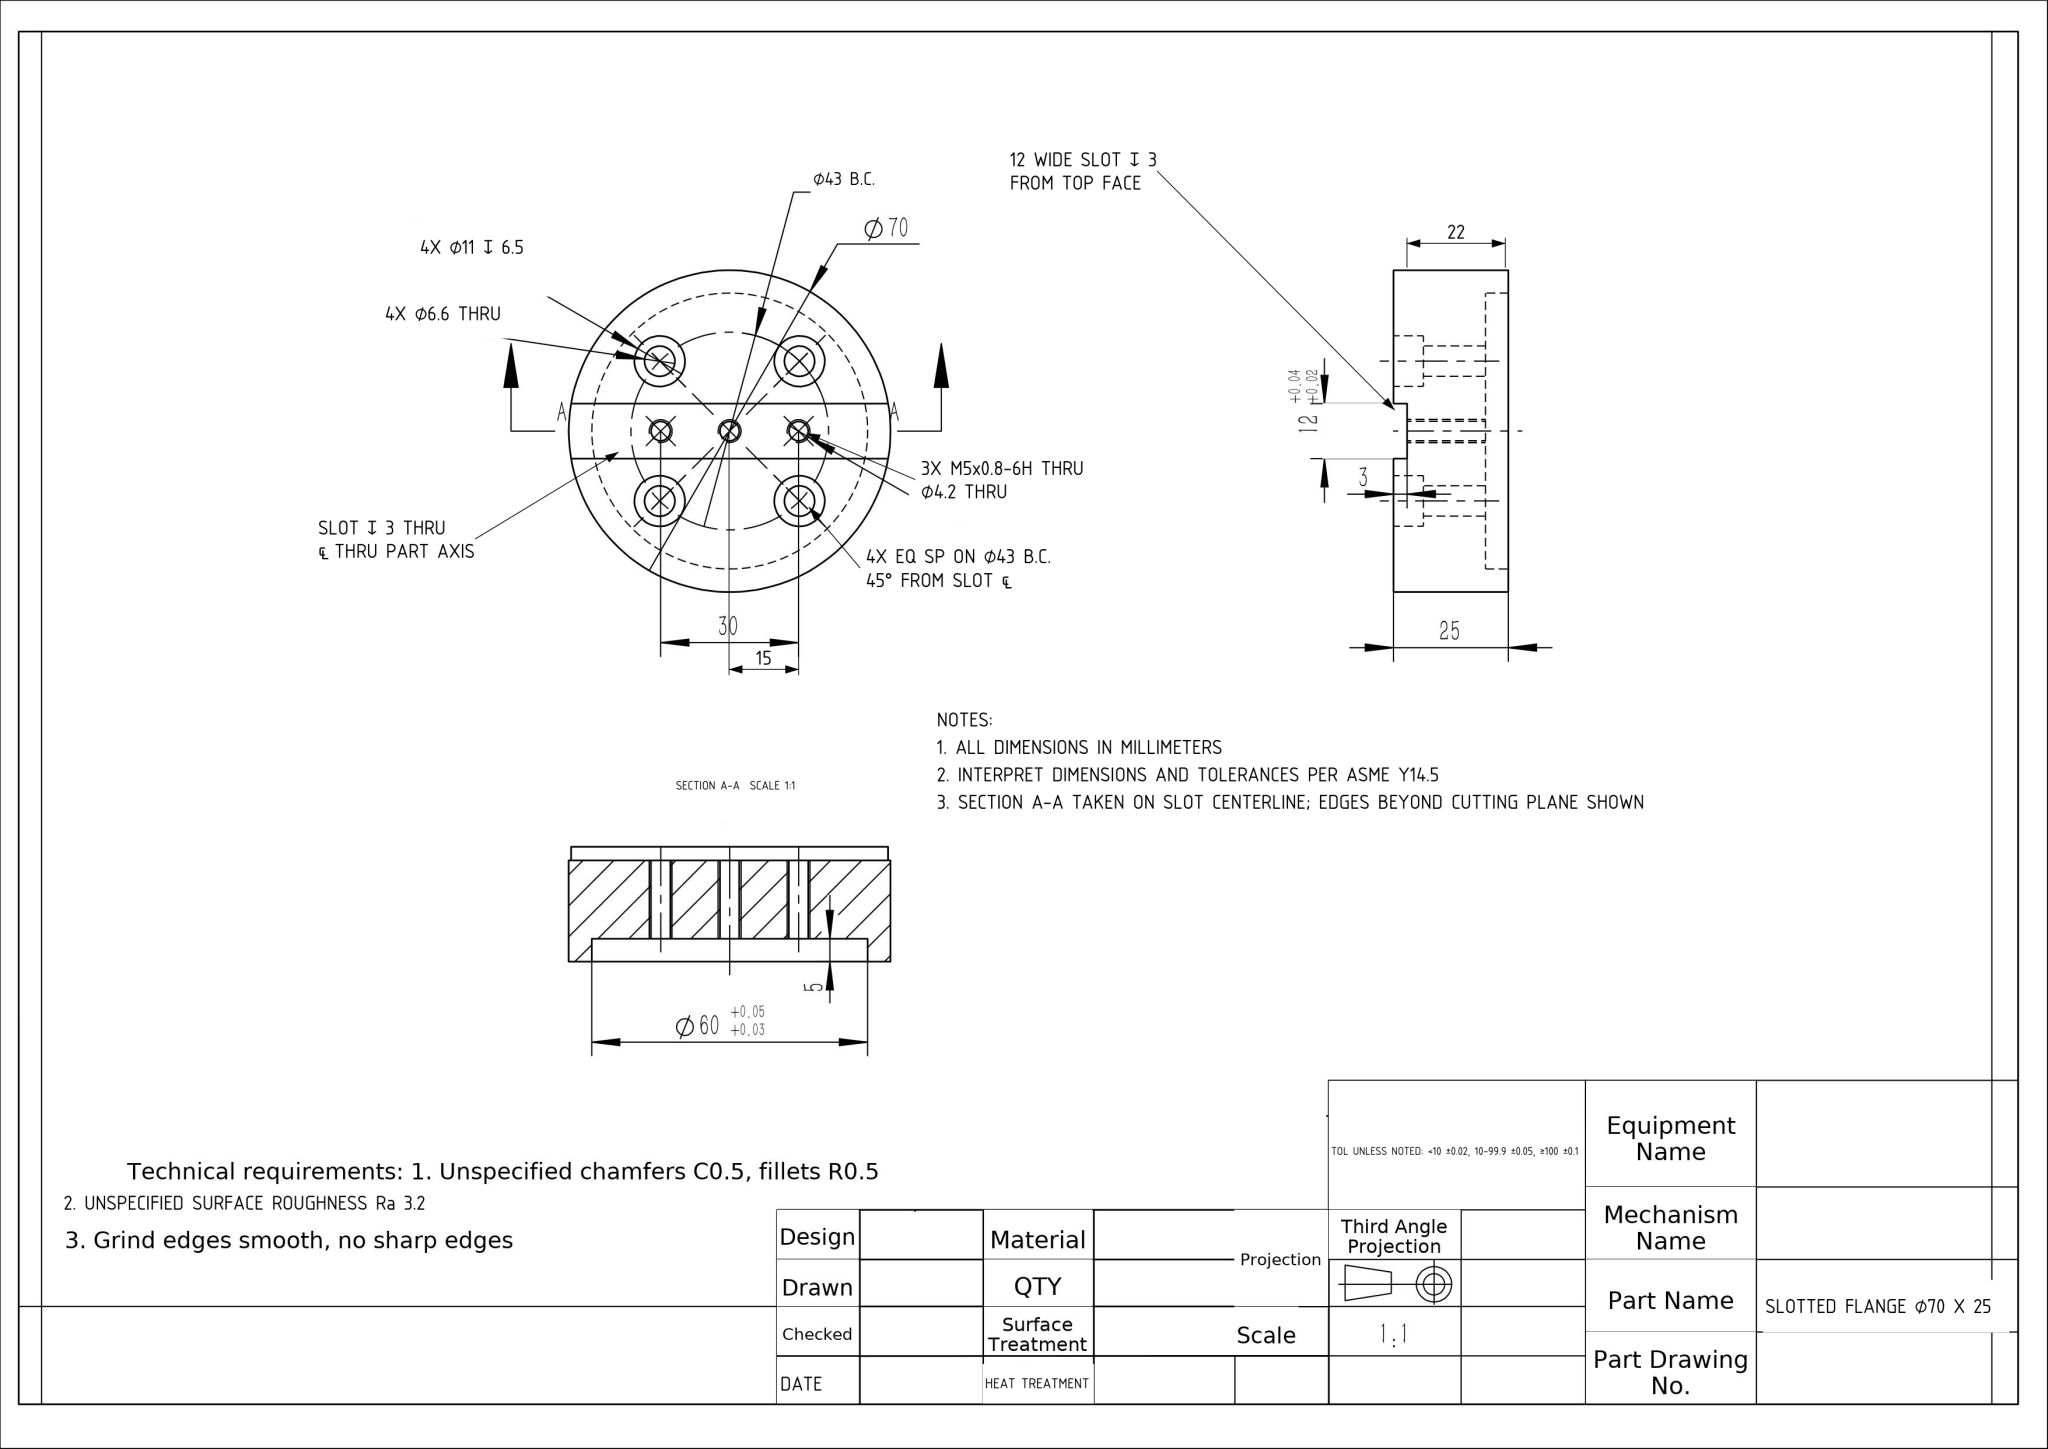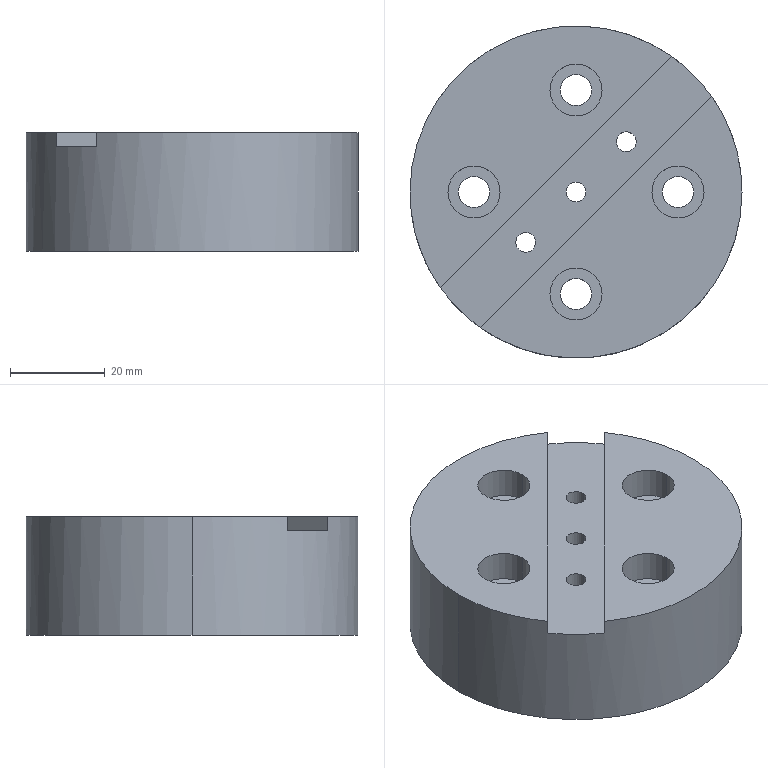Part | NX | mm | 1 solid | 37 faces | box 70 x 70 x 25 mm | volume 74542 mm3 | cylinder 26 | plane 11 | commonest cylinder face diameters 11 x8 6.6 x8 4.2 x6 60 x2 70 x2